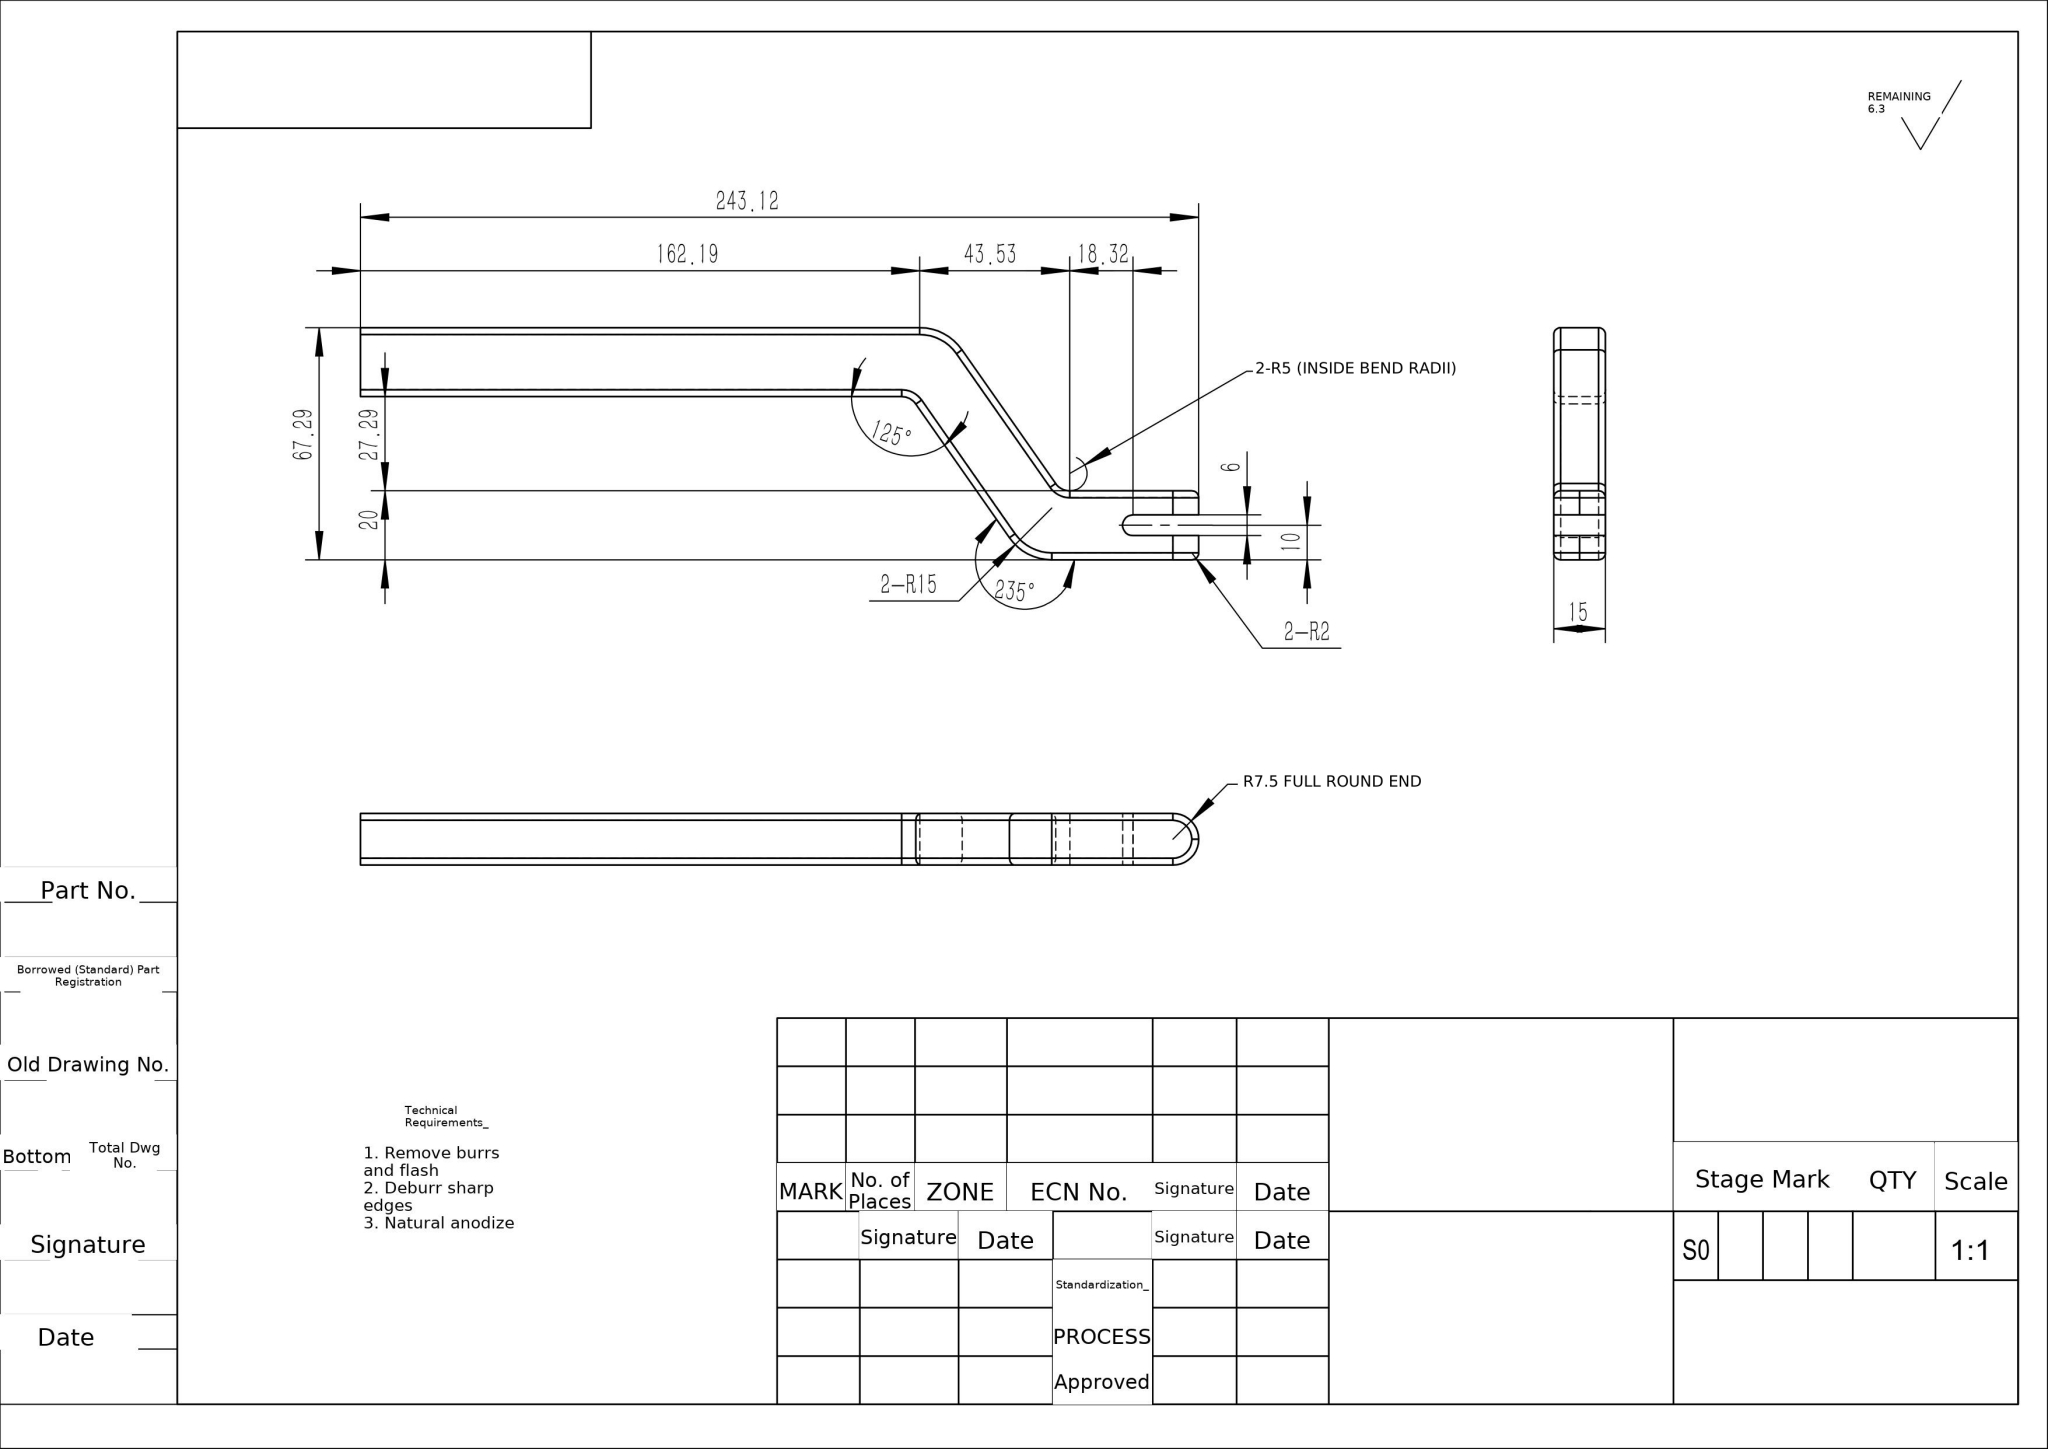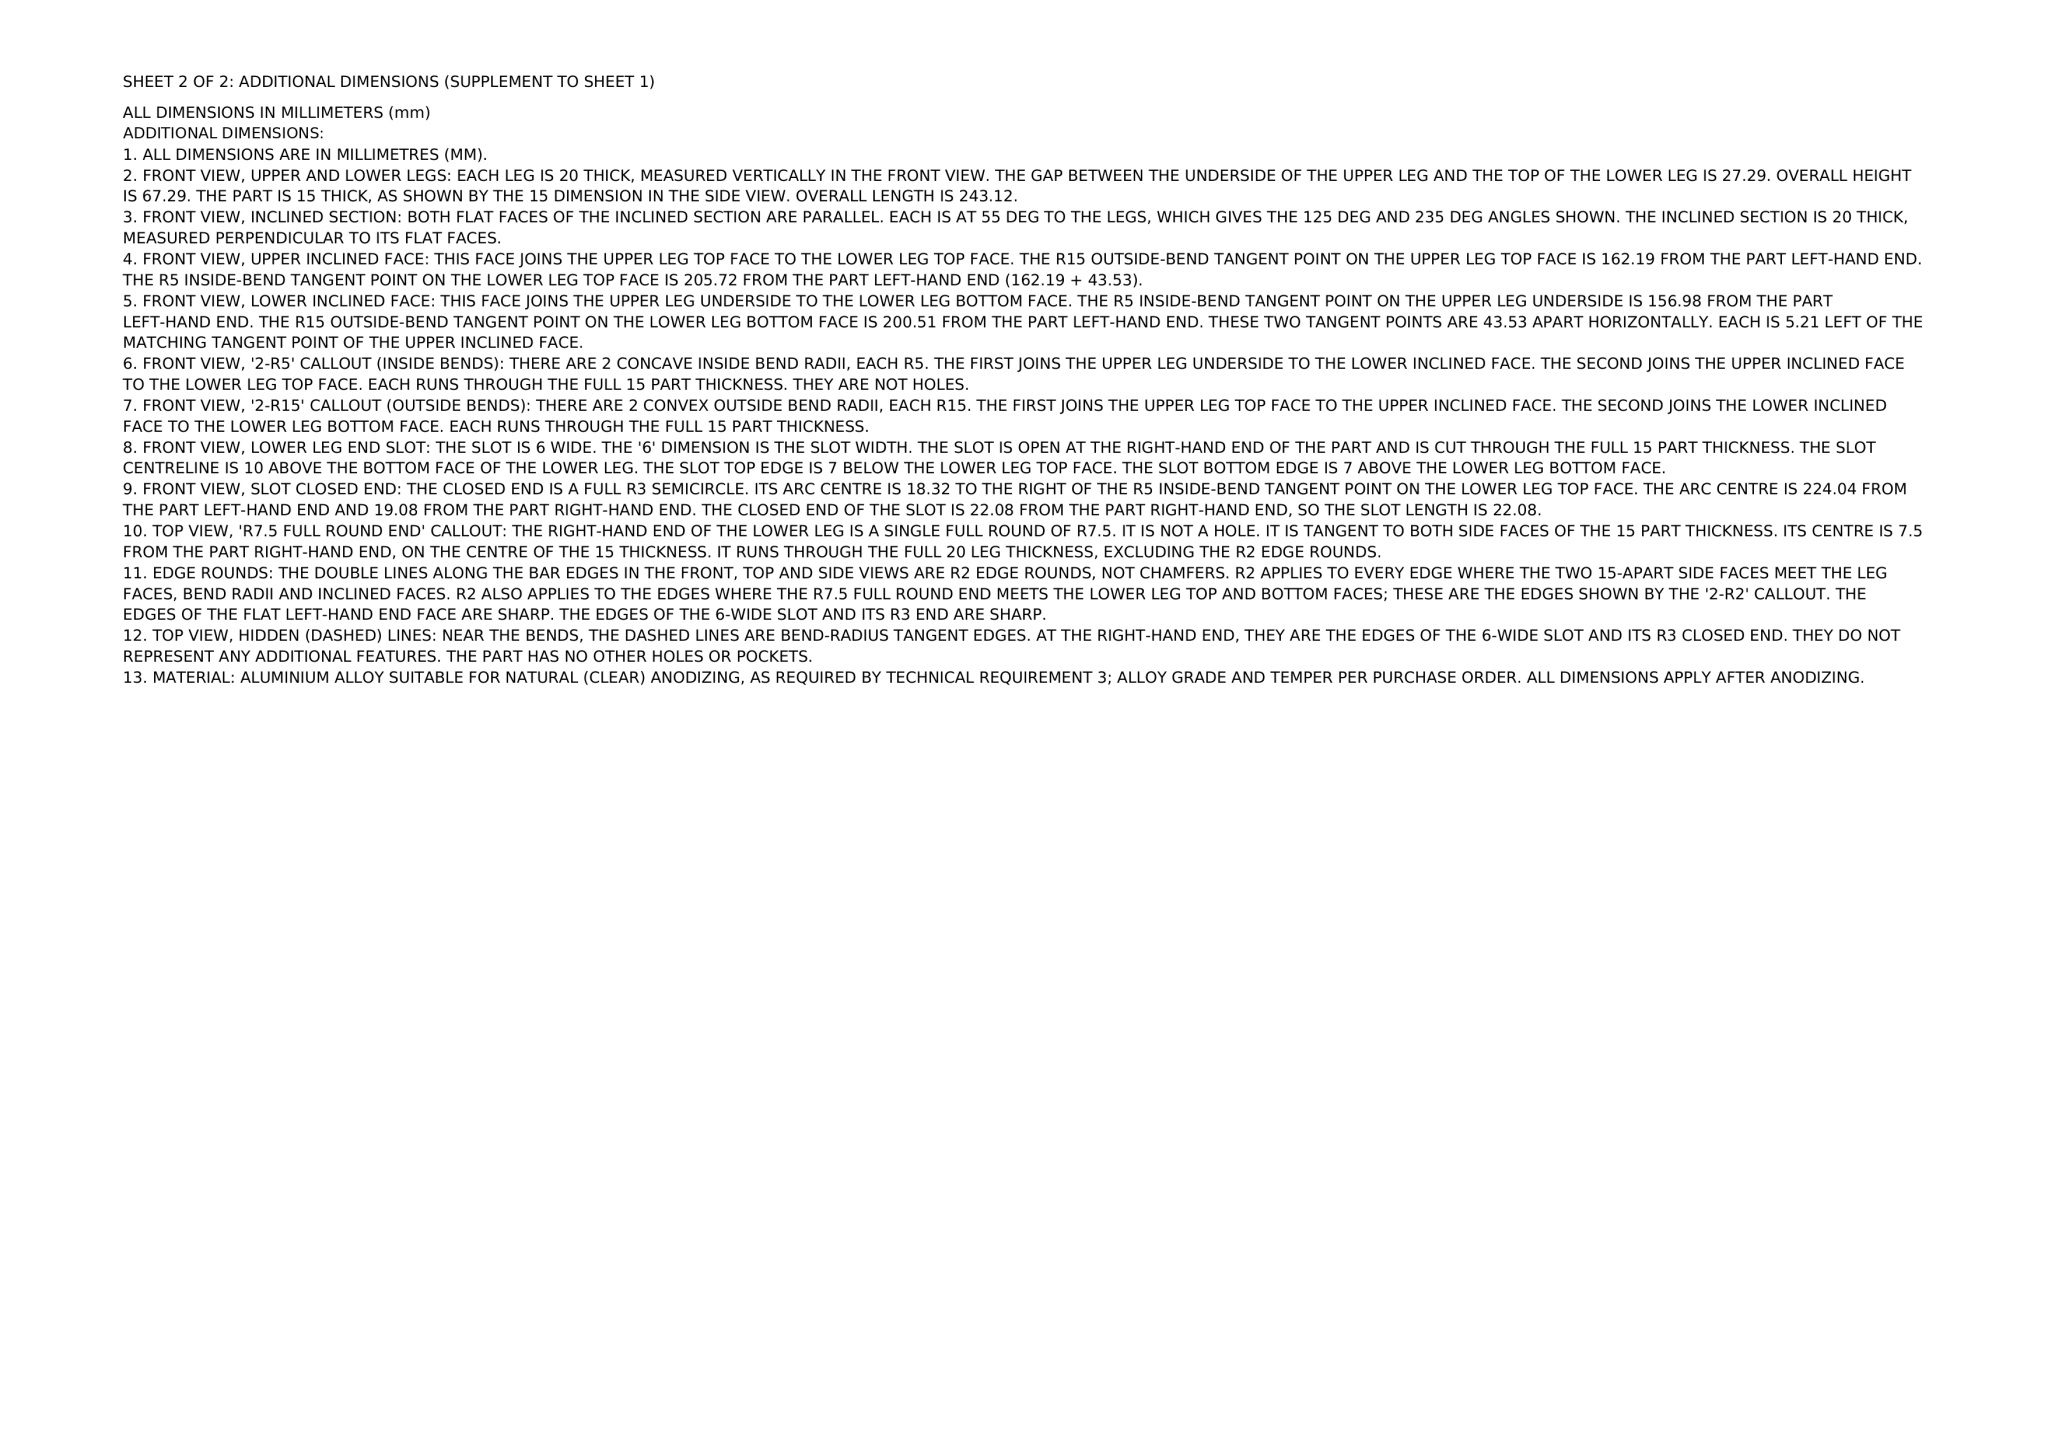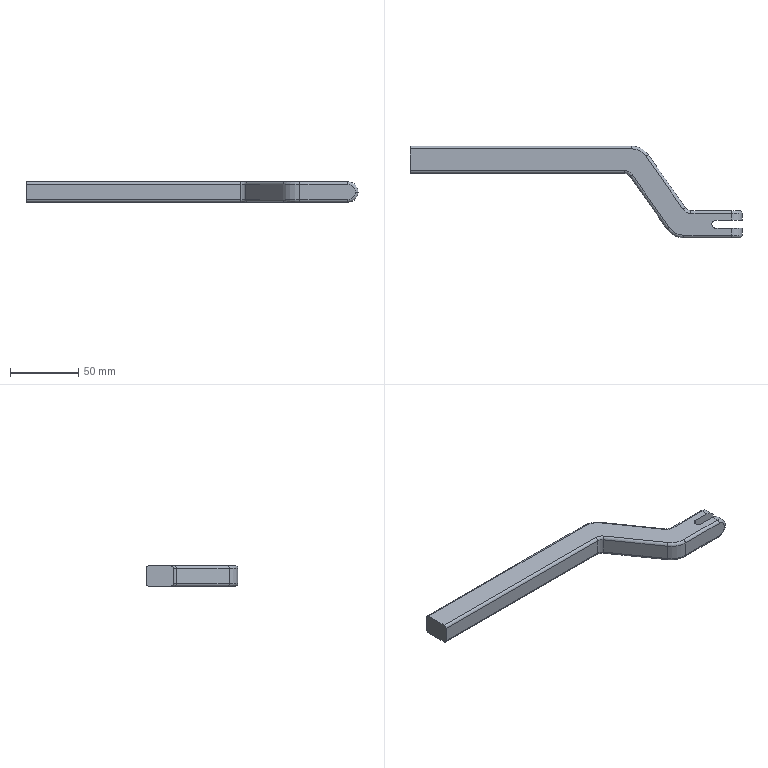Part | NX | mm | 1 solid | 44 faces | box 243.12 x 67.29 x 15 mm | volume 76884 mm3 | cylinder 21 | torus 12 | plane 11 | commonest cylinder face diameters 4 x12 15 x4 30 x2 10 x2 6 x1